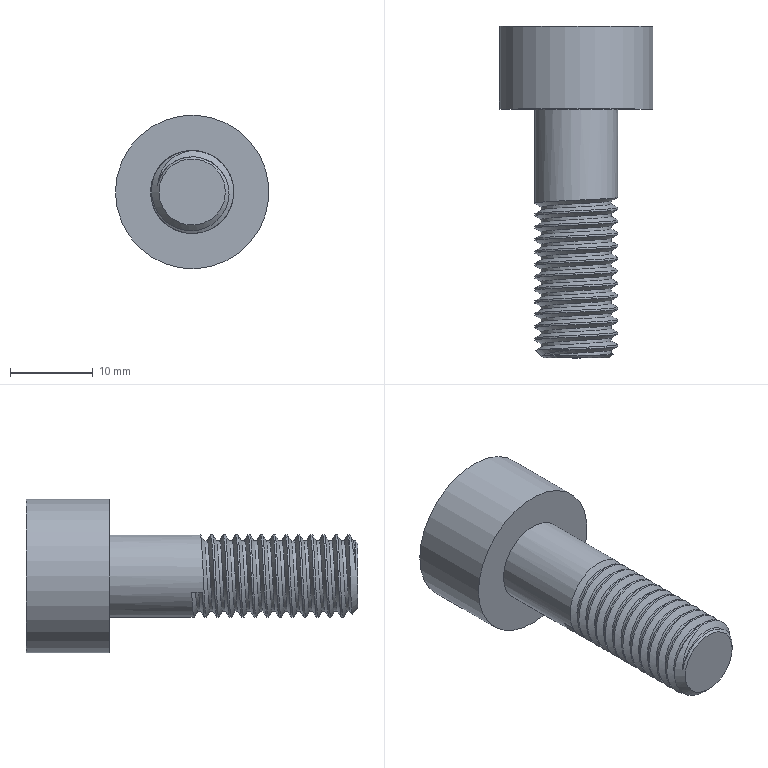Component | NX | ALLINE_SCREW_M10_3 | 1 solid | 28 faces | volume 3654 mm3 | cylinder 14 | plane 11 | spline 2 | cone 1 | commonest cylinder face diameters 10 x12 18.5 x1 8.5 x1